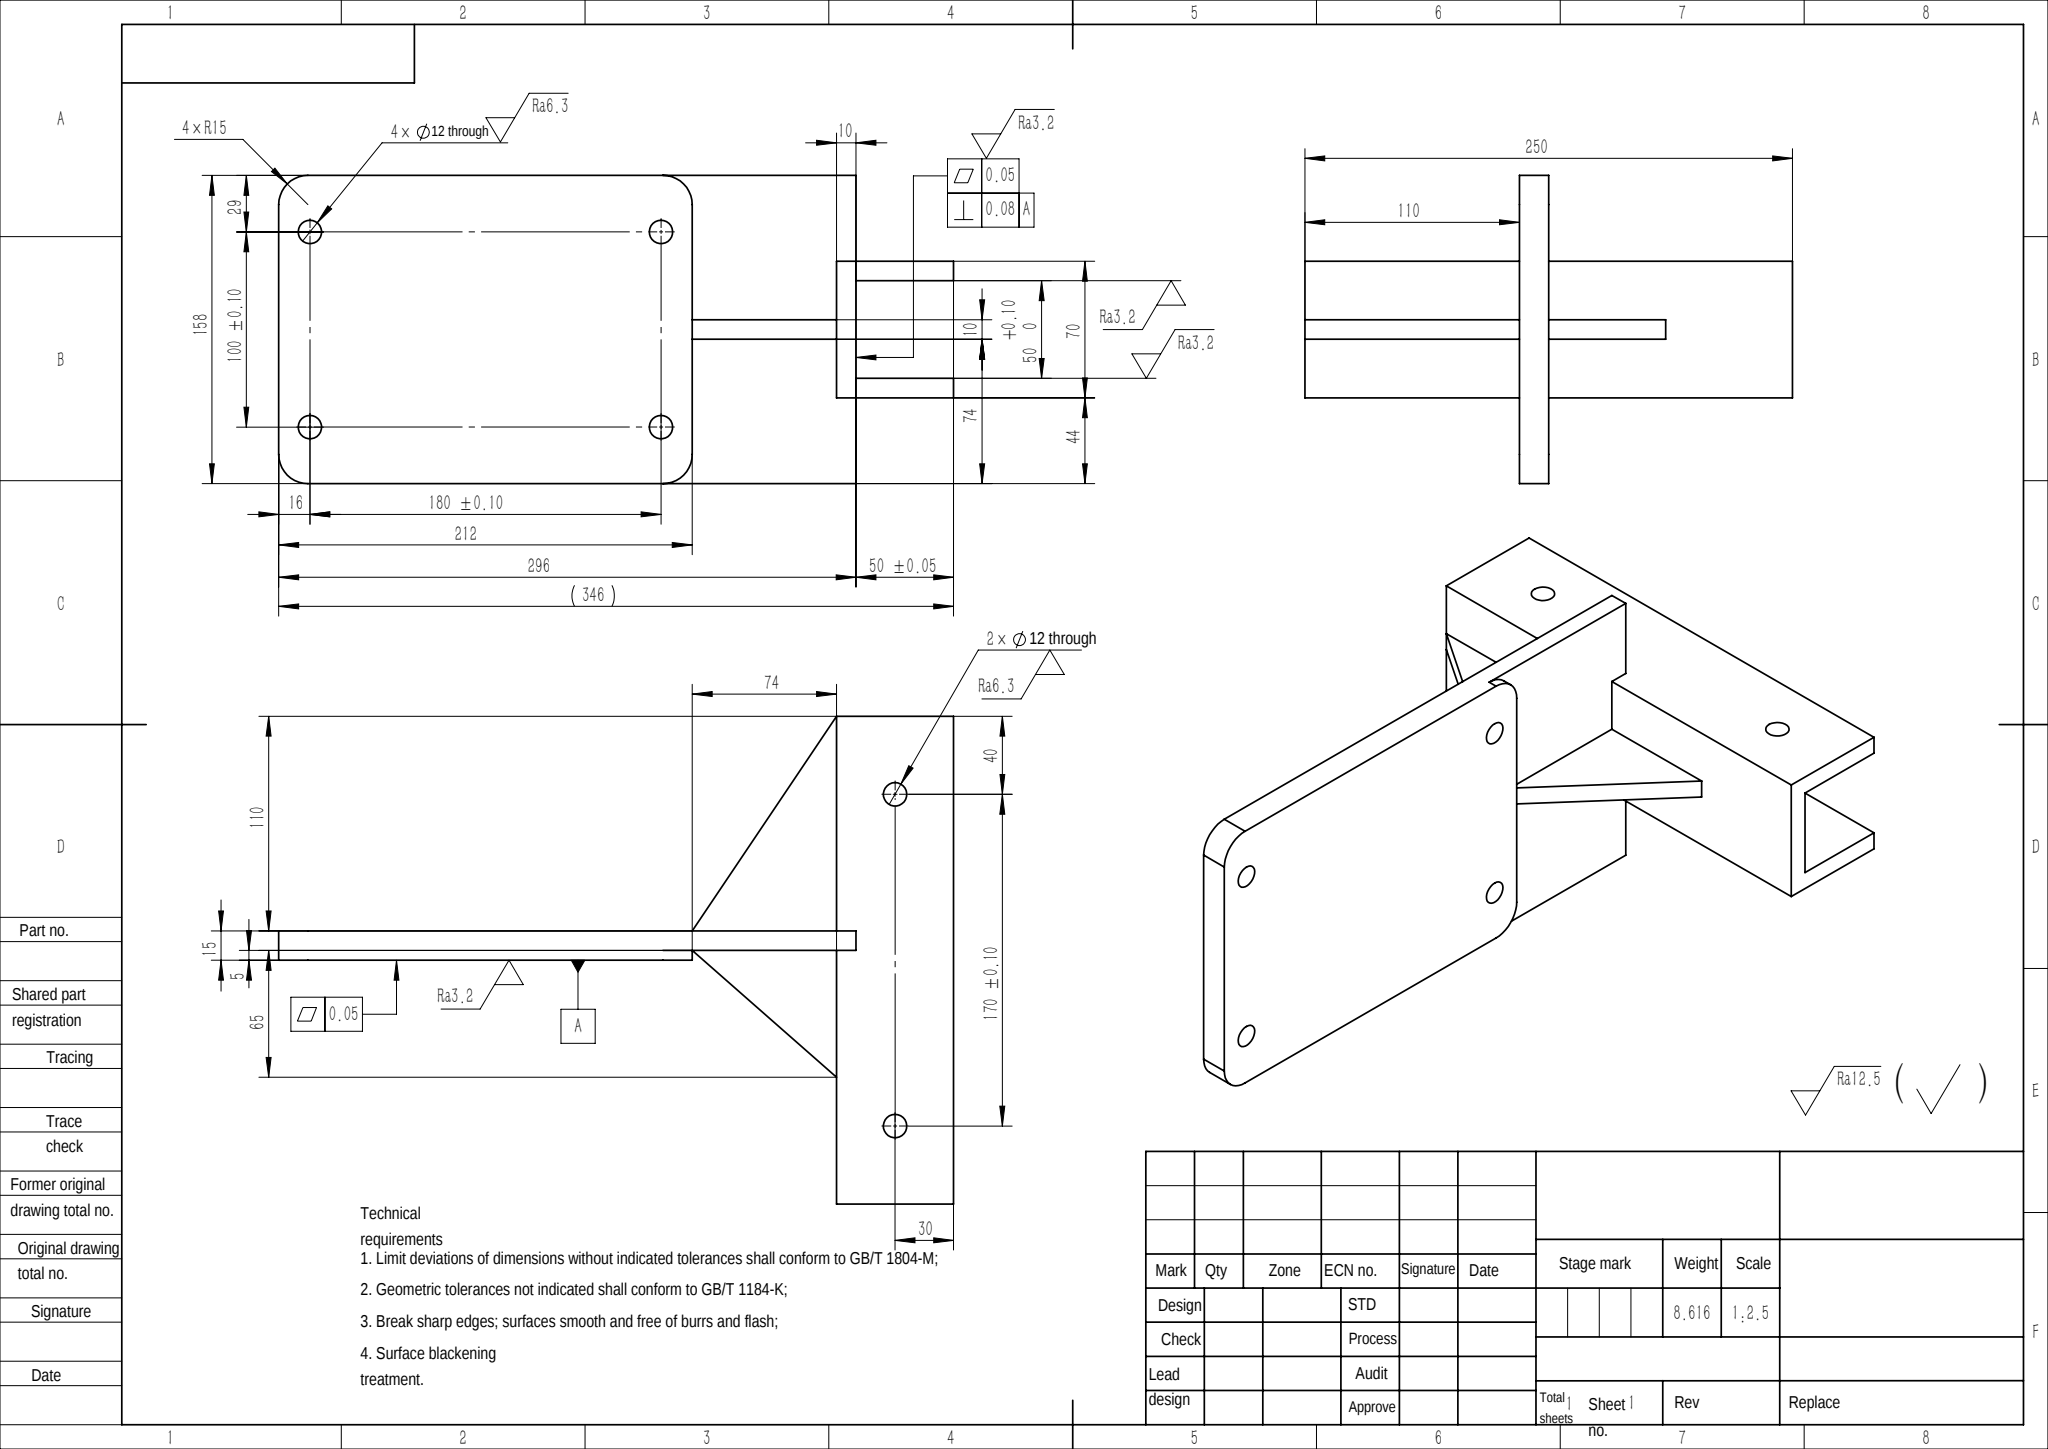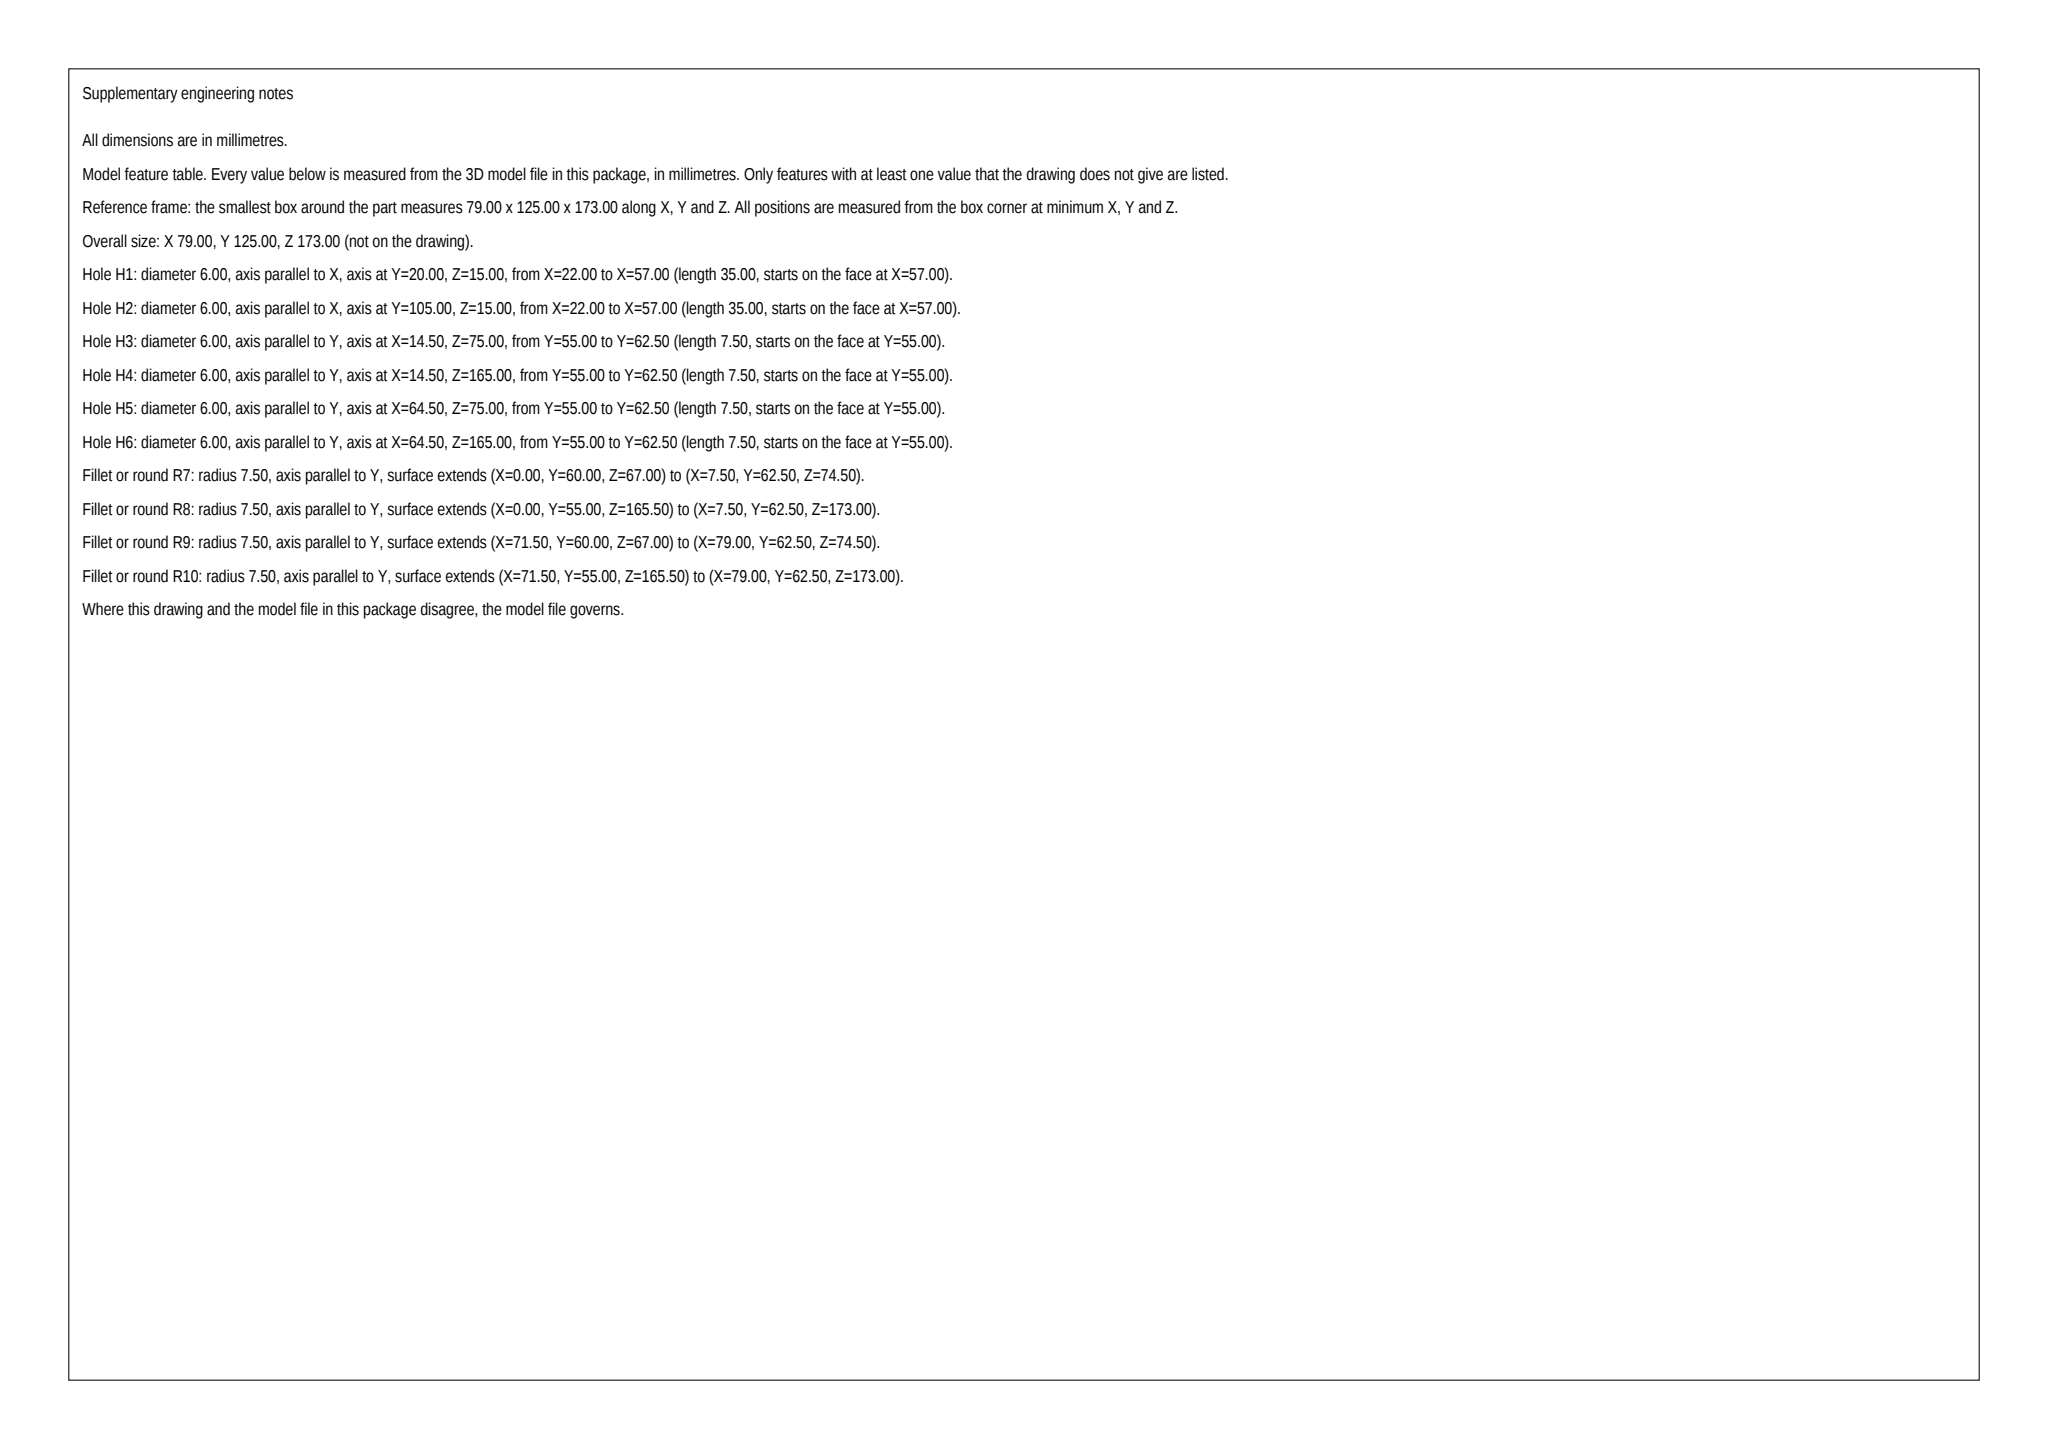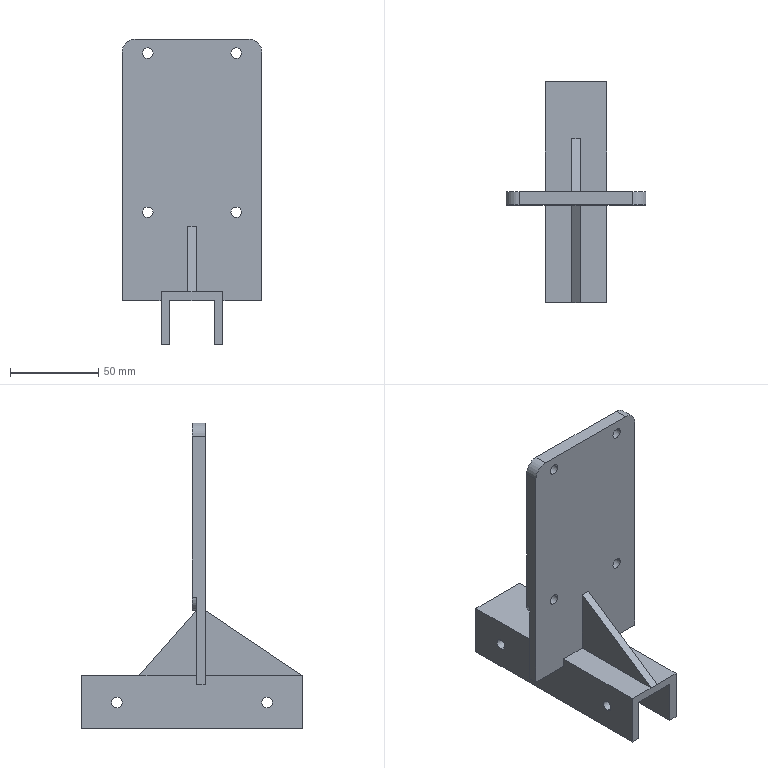Part | SolidWorks | mm | 1 solid | 48 faces | box 79 x 125 x 173 mm | volume 138084 mm3 | plane 28 | cylinder 20 | commonest cylinder face diameters 6 x16 15 x4